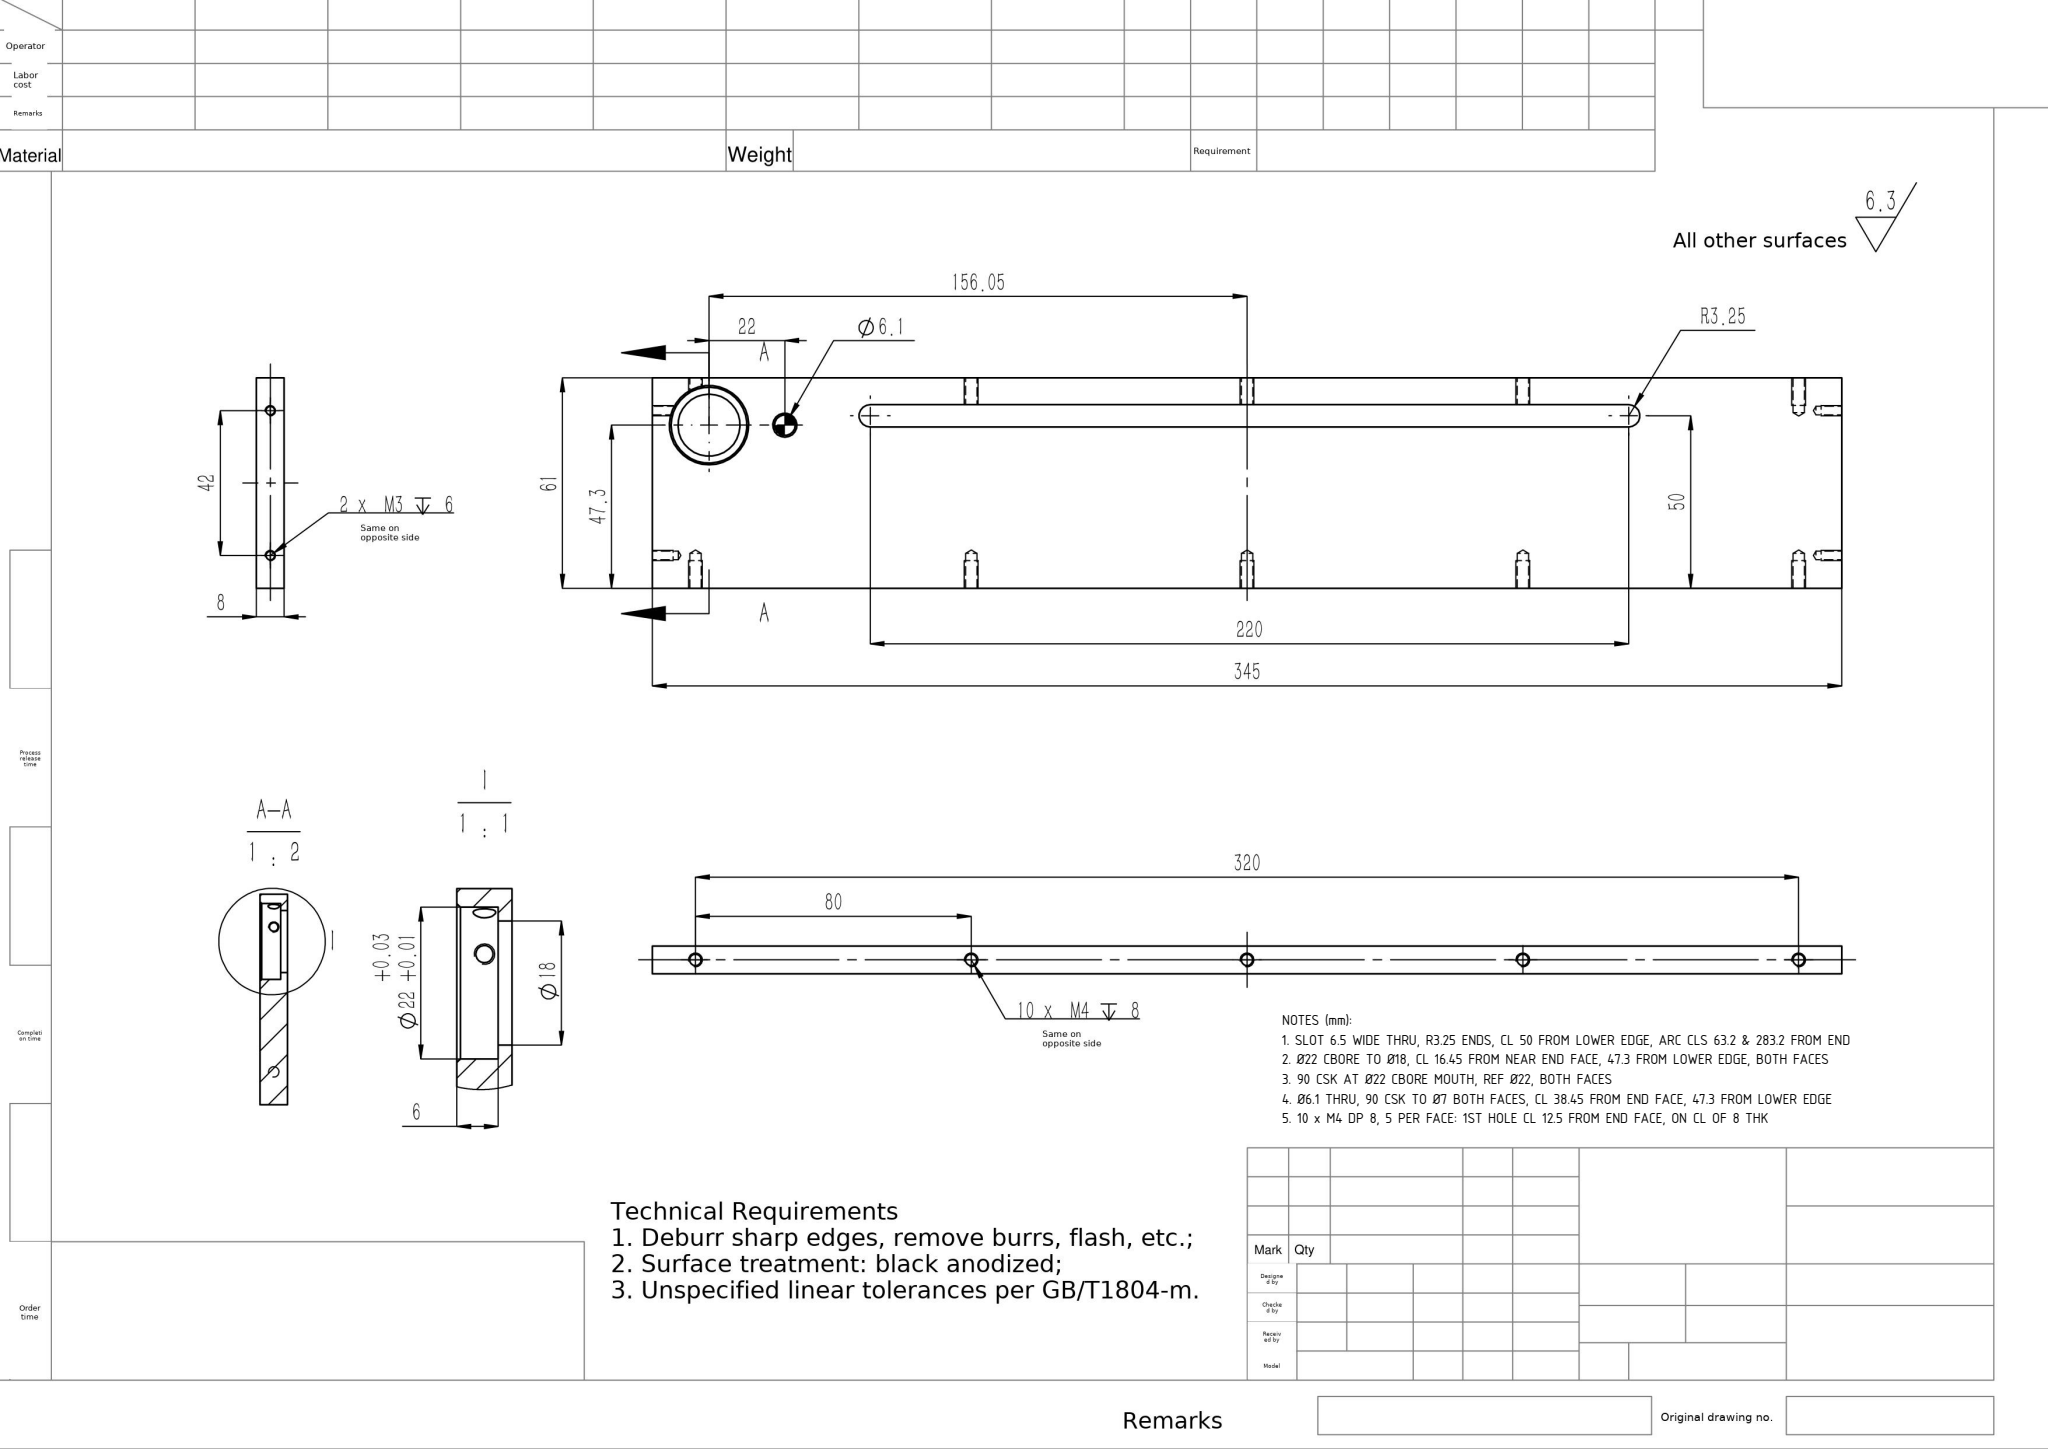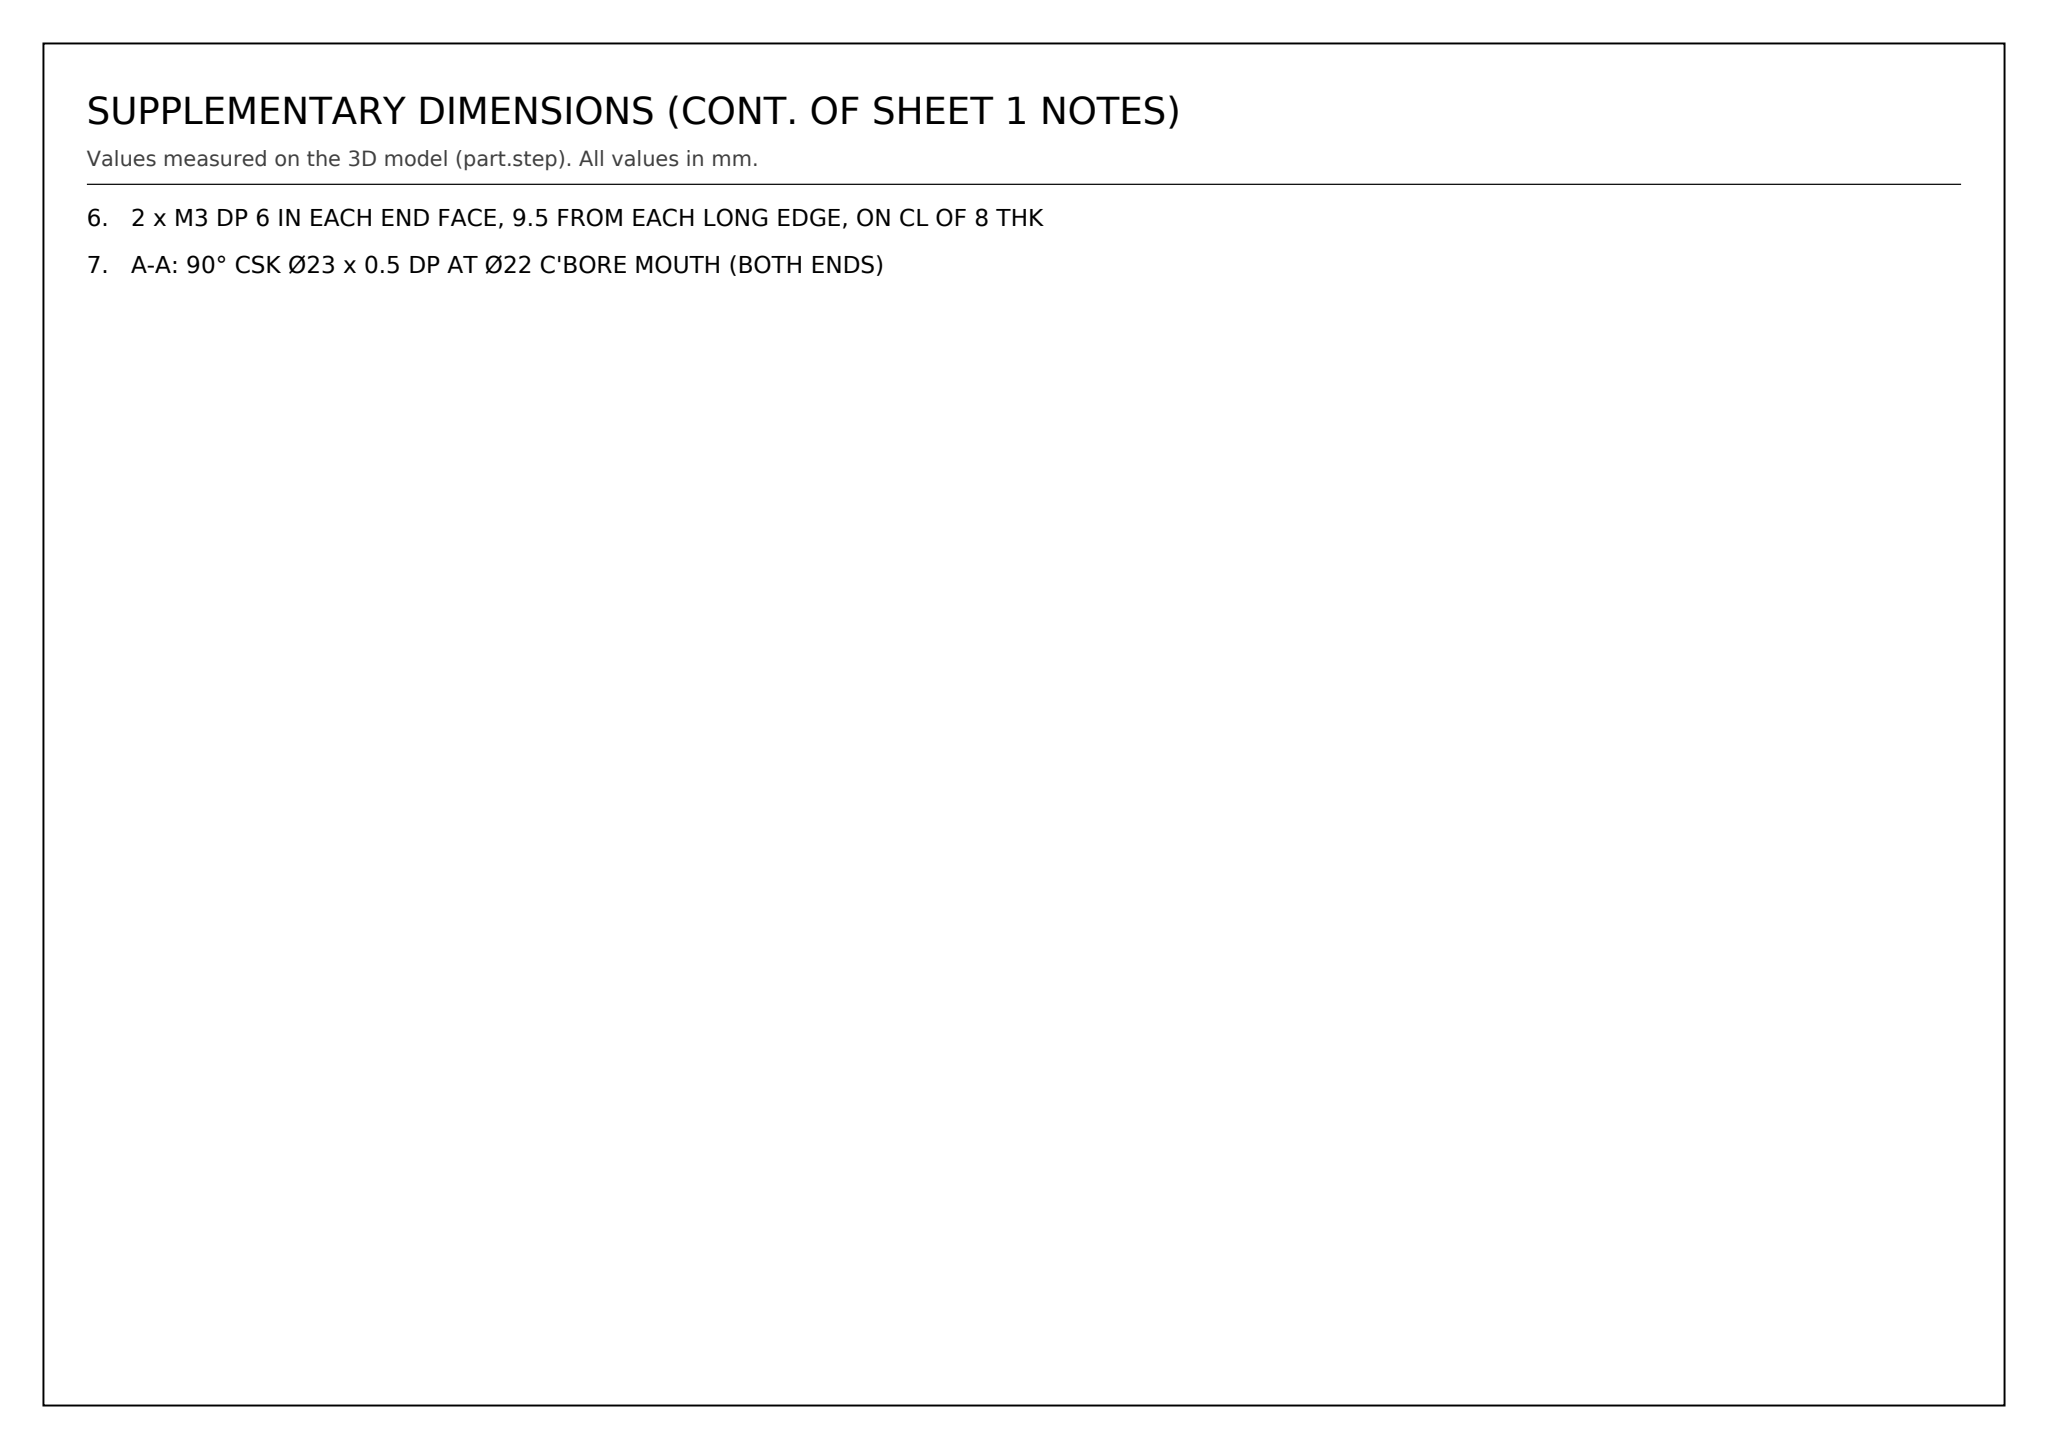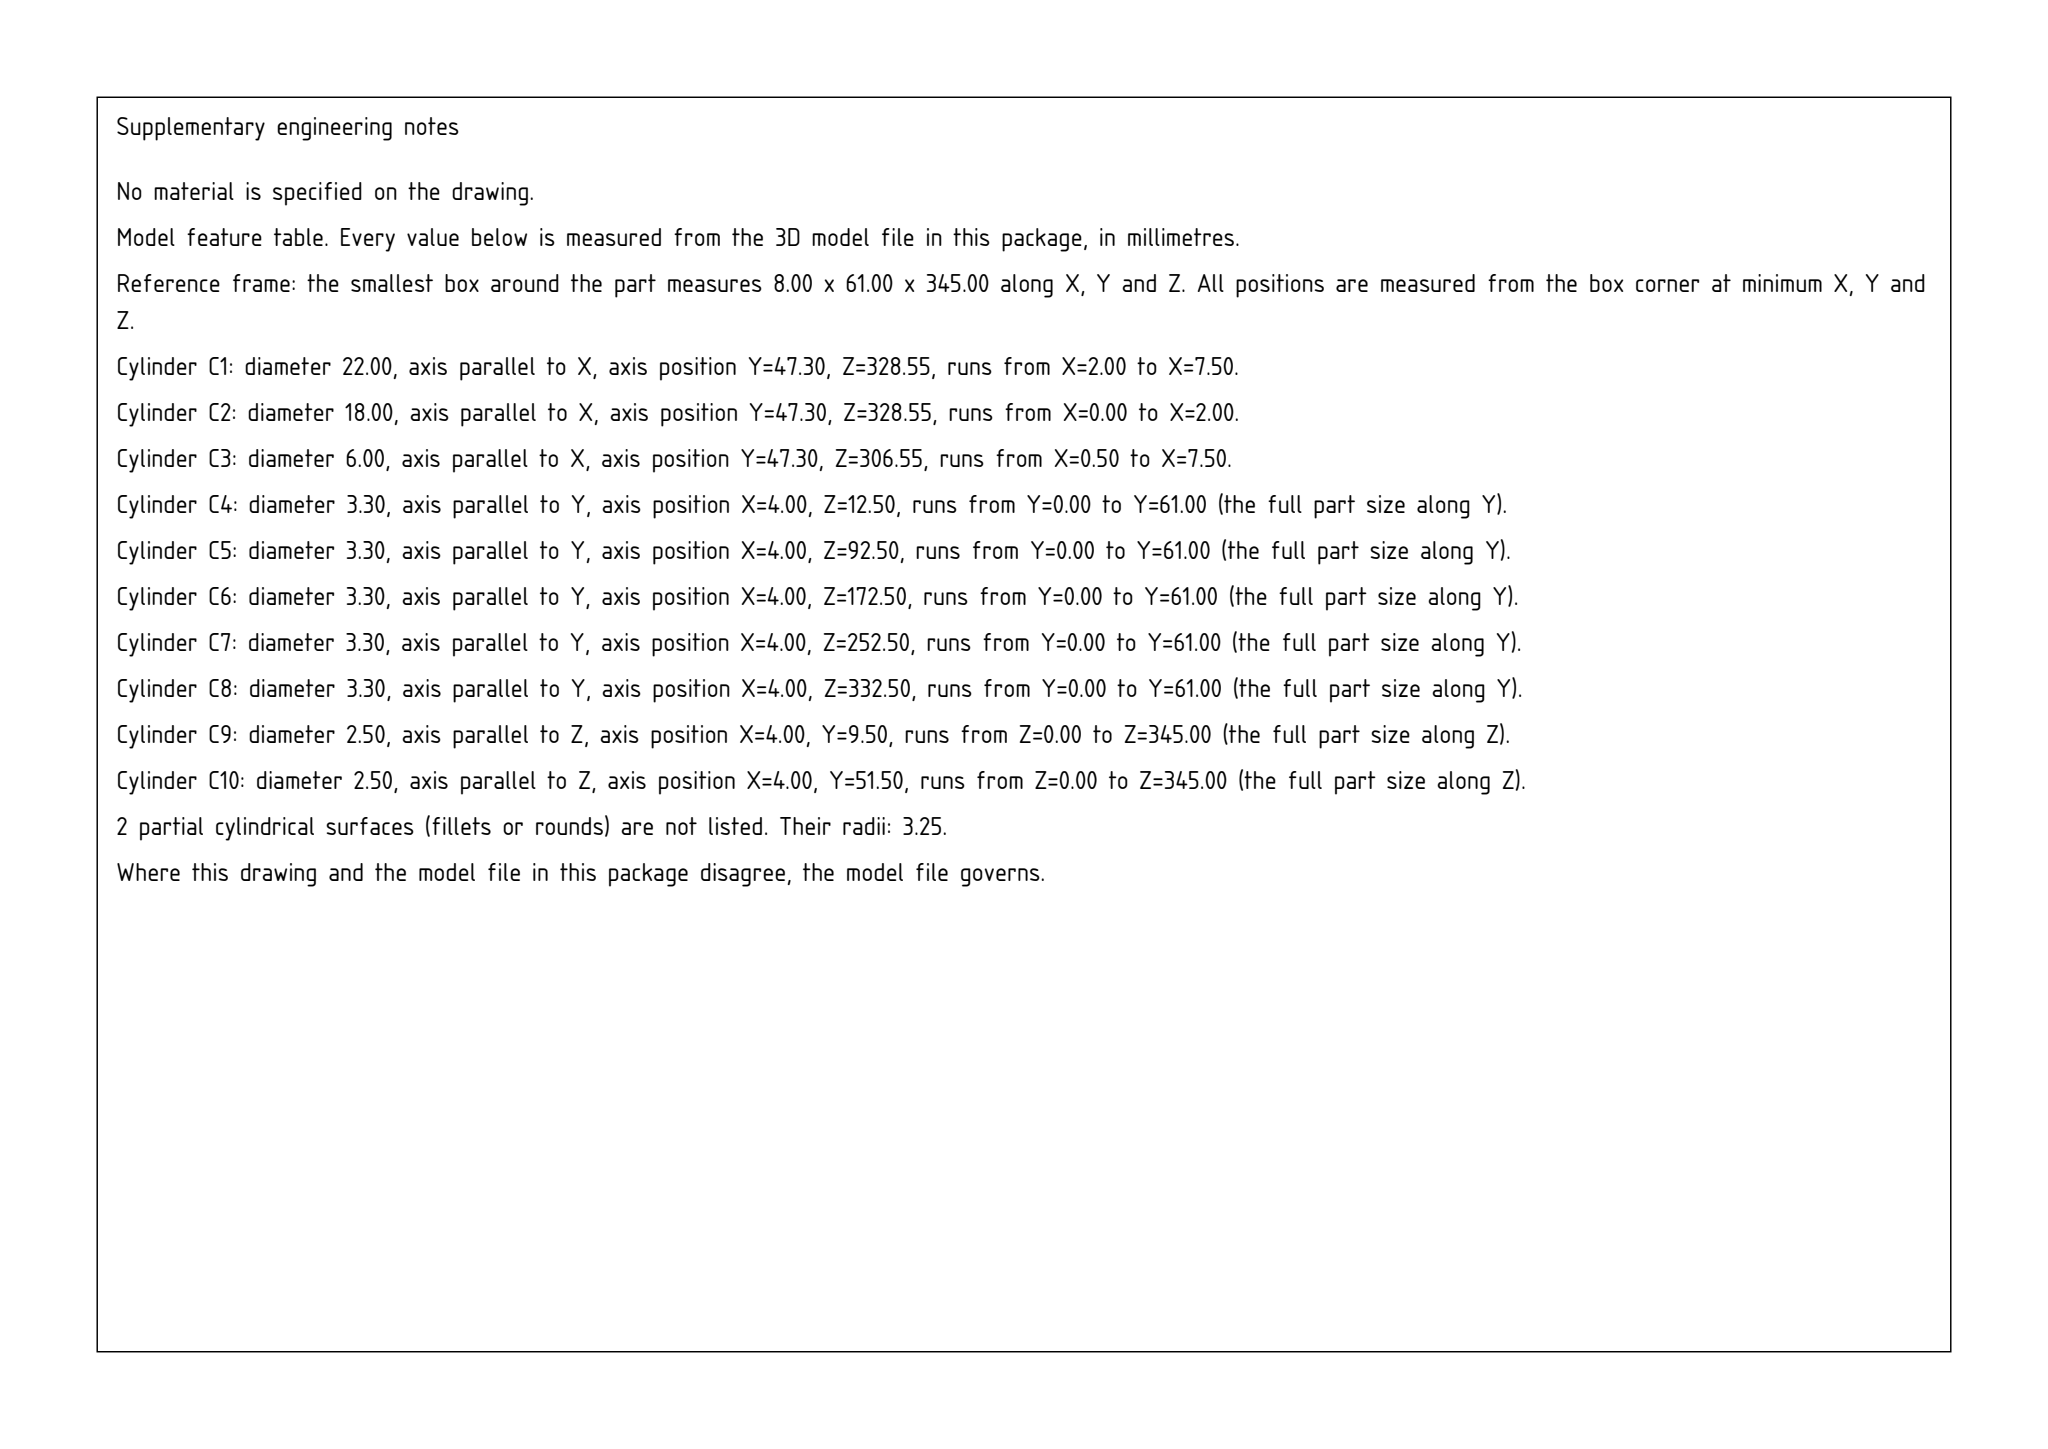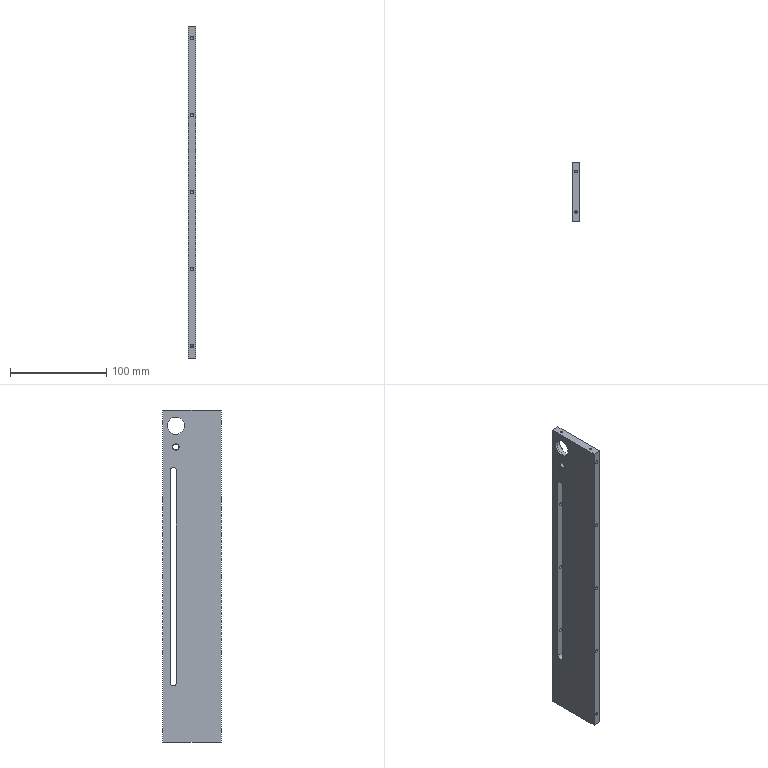Part | SolidWorks | mm | 1 solid | 69 faces | box 8 x 61 x 345 mm | volume 152716 mm3 | cylinder 36 | cone 24 | plane 9 | commonest cylinder face diameters 3.3 x20 2.5 x8 6 x2 18 x2 22 x2 6.5 x2
Drawing notes:
SLOT 6.5 WIDE THRU, R3.25 ENDS, CL 50 FROM LOWER EDGE, ARC CLS 63.2 & 283.2 FROM END | from the solid: y-planes 46.75/53.25 = 6.5 wide, CL y=50; Ø6.5 x-axis thru holes (len 8) at z=61.8 & 281.8; 345-281.8=63.2, 345-61.8=283.2
Ø22 CBORE TO Ø18, CL 16.45 FROM NEAR END FACE, 47.3 FROM LOWER EDGE, BOTH FACES | from the solid: Ø22 and Ø18 x-axis bores at y=47.3, z=328.55, 2 each; 345-328.55=16.45
90 CSK AT Ø22 CBORE MOUTH, REF Ø22, BOTH FACES | from the solid: cones[90.0, ref dia 22.0] x2 at y=47.3, z=328.55
Ø6.1 THRU, 90 CSK TO Ø7 BOTH FACES, CL 38.45 FROM END FACE, 47.3 FROM LOWER EDGE | from the solid: Ø6 x-axis hole at y=47.3, z=306.55 (345-306.55=38.45); cones 90°, ref dia 7.0 x2
10 x M4 DP 8, 5 PER FACE: 1ST HOLE CL 12.5 FROM END FACE, ON CL OF 8 THK | from the solid: Ø3.3 y-axis holes at x=4.0, z=12.5/92.5/172.5/252.5/332.5, 2 per z (both faces)
2 x M3 DP 6 IN EACH END FACE, 9.5 FROM EACH LONG EDGE, ON CL OF 8 THK | from the solid: Ø2.5 z-axis holes at x=4.0, y=9.5 & 51.5 (61-51.5=9.5), at both z=0 and z=345
A-A: 90° CSK Ø23 x 0.5 DP AT Ø22 C'BORE MOUTH (BOTH ENDS) | from the solid: cones[90°, ref_dia 22] x2 coaxial with Ø22 c'bore (pos y47.3/z328.55); plate thk 8 = 0.5 csk + 5.5 Ø22 + 2.0 Ø18, so 90° csk rises 0.5 to Ø23
build123d program:
from build123d import *

# Parameters (mm, degrees)
SKETCH1_W                  = 8
SKETCH1_H                  = 345
BOSS_EXTRUDE1_DEPTH        = 61
SKETCH2_R                  = 11
CUT_EXTRUDE1_DEPTH         = 6
SKETCH3_R                  = 9
CUT_EXTRUDE2_DEPTH         = 10
CHAMFER1_SIZE              = 0.5
SIZE_MM_DOWEL_PIN_HOLE1_D  = 6
CHAMFER2_SIZE              = 0.5
M4_TAPPED_HOLE1_AT_2_COUNT = 2
M4_TAPPED_HOLE1_AT_2_PITCH = 80
M4_TAPPED_HOLE1_AT_3_COUNT = 2
M4_TAPPED_HOLE1_AT_3_PITCH = 160
M4_TAPPED_HOLE1_AT_4_COUNT = 2
M4_TAPPED_HOLE1_AT_4_PITCH = 240
M4_TAPPED_HOLE1_AT_5_COUNT = 2
M4_TAPPED_HOLE1_AT_5_PITCH = 320
M3_TAPPED_HOLE1_AT_2_COUNT = 2
M3_TAPPED_HOLE1_AT_2_PITCH = 42
CUT_EXTRUDE3_DEPTH         = 456.121


with BuildPart() as part:
    # Sketch1 → Boss-Extrude1 (new body)
    with BuildSketch(Plane(origin=(0, -12.885, 0), x_dir=(1, 0, 0), z_dir=(0, 1, 0))):
        with Locations((-33.599, -280)):
            Rectangle(SKETCH1_W, SKETCH1_H)
    extrude(amount=BOSS_EXTRUDE1_DEPTH)

    # Sketch2 → Cut-Extrude1 (cut)
    with BuildSketch(Plane(origin=(-29.599, 0, 0), x_dir=(0, 0, -1), z_dir=(1, 0, 0))):
        with Locations(Location((-436.05, 34.415, 0), (0, 0, 90))):
            Circle(SKETCH2_R)
    extrude(amount=-CUT_EXTRUDE1_DEPTH, mode=Mode.SUBTRACT)

    # Sketch3 → Cut-Extrude2 (cut)
    with BuildSketch(Plane(origin=(-35.599, 0, 0), x_dir=(0, 0, -1), z_dir=(1, 0, 0))):
        with Locations(Location((-436.05, 34.415, 0), (0, 0, 90))):
            Circle(SKETCH3_R)
    extrude(amount=-CUT_EXTRUDE2_DEPTH, mode=Mode.SUBTRACT)

    # Chamfer1
    chamfer1_edges = [part.edges().sort_by_distance(p)[0] for p in [
        (-29.599, 23.415, 436.05),
    ]]
    chamfer(chamfer1_edges, length=CHAMFER1_SIZE)

    # Size mm Dowel Pin Hole1 (through all)
    with Locations(Plane(origin=(-29.599, 0, 0), x_dir=(0, 0, -1), z_dir=(1, 0, 0))):
        with Locations((-414.05, 34.415)):
            Hole(SIZE_MM_DOWEL_PIN_HOLE1_D / 2)

    # Chamfer2
    chamfer2_edges = [part.edges().sort_by_distance(p)[0] for p in [
        (-29.599, 34.415, 411.05),
        (-37.599, 34.415, 411.05),
    ]]
    chamfer(chamfer2_edges, length=CHAMFER2_SIZE)

    # Sketch7 → M4 Tapped Hole1 (revolve, cut)
    with BuildSketch(Plane(origin=(-33.599, -12.885, 440), x_dir=(0, 0, -1), z_dir=(1, 0, 0))):
        Polygon((0, 0), (0, 11.091), (1.65, 10.1), (1.65, 0), align=None)
    m4_tapped_hole1 = revolve(axis=Axis((-33.599, -19.235, 440), (0, 1, 0)), mode=Mode.SUBTRACT)

    # M4 Tapped Hole1 at 2: M4 Tapped Hole1 ×2
    with Locations(*[(0, 0, -i * M4_TAPPED_HOLE1_AT_2_PITCH) for i in range(1, M4_TAPPED_HOLE1_AT_2_COUNT)]):
        add(m4_tapped_hole1, mode=Mode.SUBTRACT)

    # M4 Tapped Hole1 at 3: M4 Tapped Hole1 ×2
    with Locations(*[(0, 0, -i * M4_TAPPED_HOLE1_AT_3_PITCH) for i in range(1, M4_TAPPED_HOLE1_AT_3_COUNT)]):
        add(m4_tapped_hole1, mode=Mode.SUBTRACT)

    # M4 Tapped Hole1 at 4: M4 Tapped Hole1 ×2
    with Locations(*[(0, 0, -i * M4_TAPPED_HOLE1_AT_4_PITCH) for i in range(1, M4_TAPPED_HOLE1_AT_4_COUNT)]):
        add(m4_tapped_hole1, mode=Mode.SUBTRACT)

    # M4 Tapped Hole1 at 5: M4 Tapped Hole1 ×2
    with Locations(*[(0, 0, -i * M4_TAPPED_HOLE1_AT_5_PITCH) for i in range(1, M4_TAPPED_HOLE1_AT_5_COUNT)]):
        add(m4_tapped_hole1, mode=Mode.SUBTRACT)

    # Sketch9 → M3 Tapped Hole1 (revolve, cut)
    with BuildSketch(Plane(origin=(-33.599, 38.615, 452.5), x_dir=(0, -1, 0), z_dir=(1, 0, 0))):
        Polygon((0, 0), (0, 8.251), (1.25, 7.5), (1.25, 0), align=None)
    m3_tapped_hole1 = revolve(axis=Axis((-33.599, 38.615, 458.85), (0, 0, -1)), mode=Mode.SUBTRACT)

    # M3 Tapped Hole1 at 2: M3 Tapped Hole1 ×2
    with Locations(*[(0, -i * M3_TAPPED_HOLE1_AT_2_PITCH, 0) for i in range(1, M3_TAPPED_HOLE1_AT_2_COUNT)]):
        add(m3_tapped_hole1, mode=Mode.SUBTRACT)

    # Sketch10 → Cut-Extrude3 (cut, through all)
    with BuildSketch(Plane(origin=(-29.599, 0, 0), x_dir=(0, 0, -1), z_dir=(1, 0, 0))):
        with BuildLine():
            Line((-389.3, 40.365), (-169.3, 40.365))
            ThreePointArc((-169.3, 40.365), (-166.05, 37.115), (-169.3, 33.865))
            Line((-169.3, 33.865), (-389.3, 33.865))
            ThreePointArc((-389.3, 33.865), (-392.55, 37.115), (-389.3, 40.365))
        make_face()
    extrude(amount=-CUT_EXTRUDE3_DEPTH, mode=Mode.SUBTRACT)

    # Mirror1: M3 Tapped Hole1 across plane
    add(m3_tapped_hole1.mirror(Plane.XY.offset(280)), mode=Mode.SUBTRACT)

    # Mirror1 copy 1 sketch → Mirror1 copy 1 (revolve, cut)
    with BuildSketch(Plane(origin=(-33.599, -3.385, 107.5), x_dir=(0, -1, 0), z_dir=(1, 0, 0))):
        Polygon((0, 0), (0, -8.251), (1.25, -7.5), (1.25, 0), align=None)
    revolve(axis=Axis((-33.599, -3.385, 101.15), (0, 0, -1)), mode=Mode.SUBTRACT)

    # Mirror2: M4 Tapped Hole1 across plane
    add(m4_tapped_hole1.mirror(Plane(origin=(0, 17.615, 0), x_dir=(0, 0, 1), z_dir=(0, -1, 0))), mode=Mode.SUBTRACT)

    # Mirror2 copy 1 sketch → Mirror2 copy 1 (revolve, cut)
    with BuildSketch(Plane(origin=(-33.599, 48.115, 360), x_dir=(0, 0, -1), z_dir=(1, 0, 0))):
        Polygon((0, 0), (0, -11.091), (1.65, -10.1), (1.65, 0), align=None)
    revolve(axis=Axis((-33.599, 54.465, 360), (0, 1, 0)), mode=Mode.SUBTRACT)

    # Mirror2 copy 2 sketch → Mirror2 copy 2 (revolve, cut)
    with BuildSketch(Plane(origin=(-33.599, 48.115, 280), x_dir=(0, 0, -1), z_dir=(1, 0, 0))):
        Polygon((0, 0), (0, -11.091), (1.65, -10.1), (1.65, 0), align=None)
    revolve(axis=Axis((-33.599, 54.465, 280), (0, 1, 0)), mode=Mode.SUBTRACT)

    # Mirror2 copy 3 sketch → Mirror2 copy 3 (revolve, cut)
    with BuildSketch(Plane(origin=(-33.599, 48.115, 200), x_dir=(0, 0, -1), z_dir=(1, 0, 0))):
        Polygon((0, 0), (0, -11.091), (1.65, -10.1), (1.65, 0), align=None)
    revolve(axis=Axis((-33.599, 54.465, 200), (0, 1, 0)), mode=Mode.SUBTRACT)

    # Mirror2 copy 4 sketch → Mirror2 copy 4 (revolve, cut)
    with BuildSketch(Plane(origin=(-33.599, 48.115, 120), x_dir=(0, 0, -1), z_dir=(1, 0, 0))):
        Polygon((0, 0), (0, -11.091), (1.65, -10.1), (1.65, 0), align=None)
    revolve(axis=Axis((-33.599, 54.465, 120), (0, 1, 0)), mode=Mode.SUBTRACT)


solid = part.part